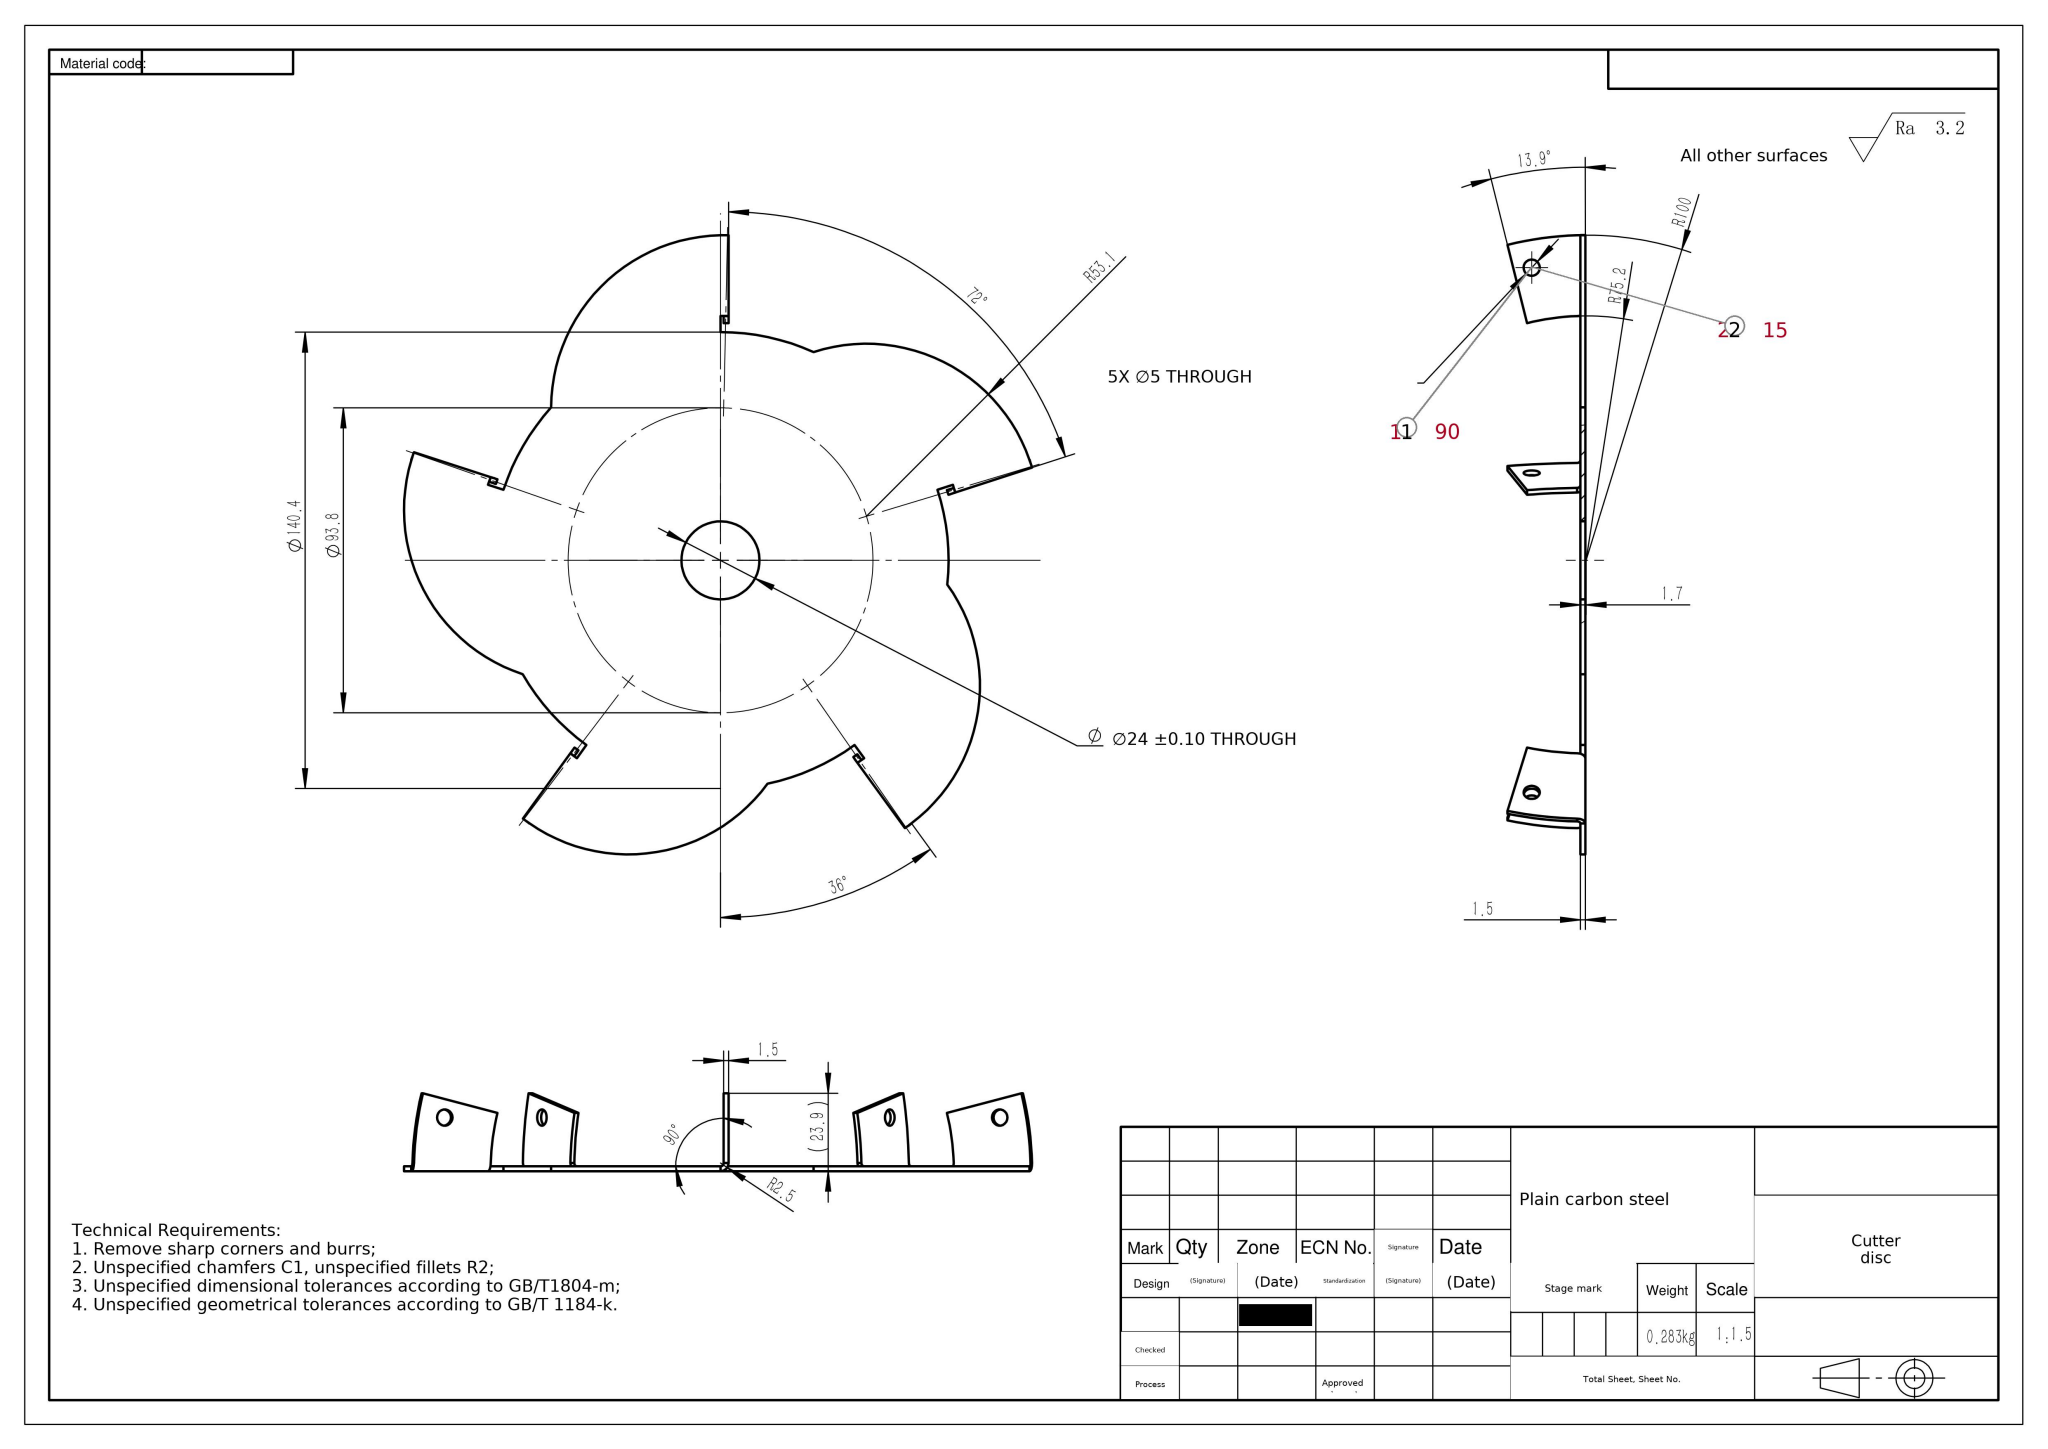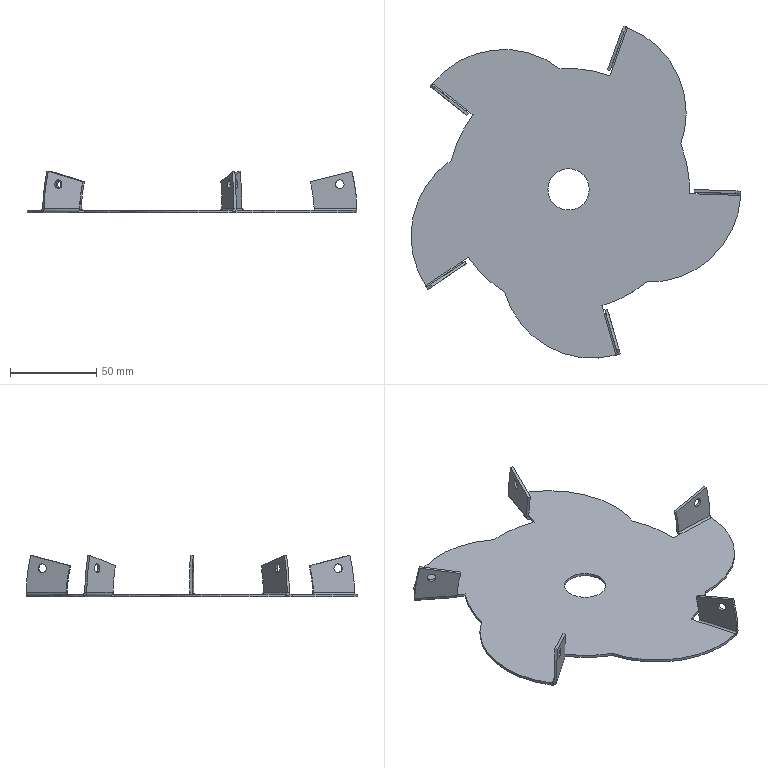Part | SolidWorks | mm | material Plain carbon steel | 1 solid | 85 faces | box 191.38 x 192.66 x 23.94 mm | volume 36247 mm3 | cylinder 43 | plane 22 | spline 20 | commonest cylinder face diameters 5 x15 106.165 x6 140.357 x5 2 x5 200 x5 150.357 x5 24 x2